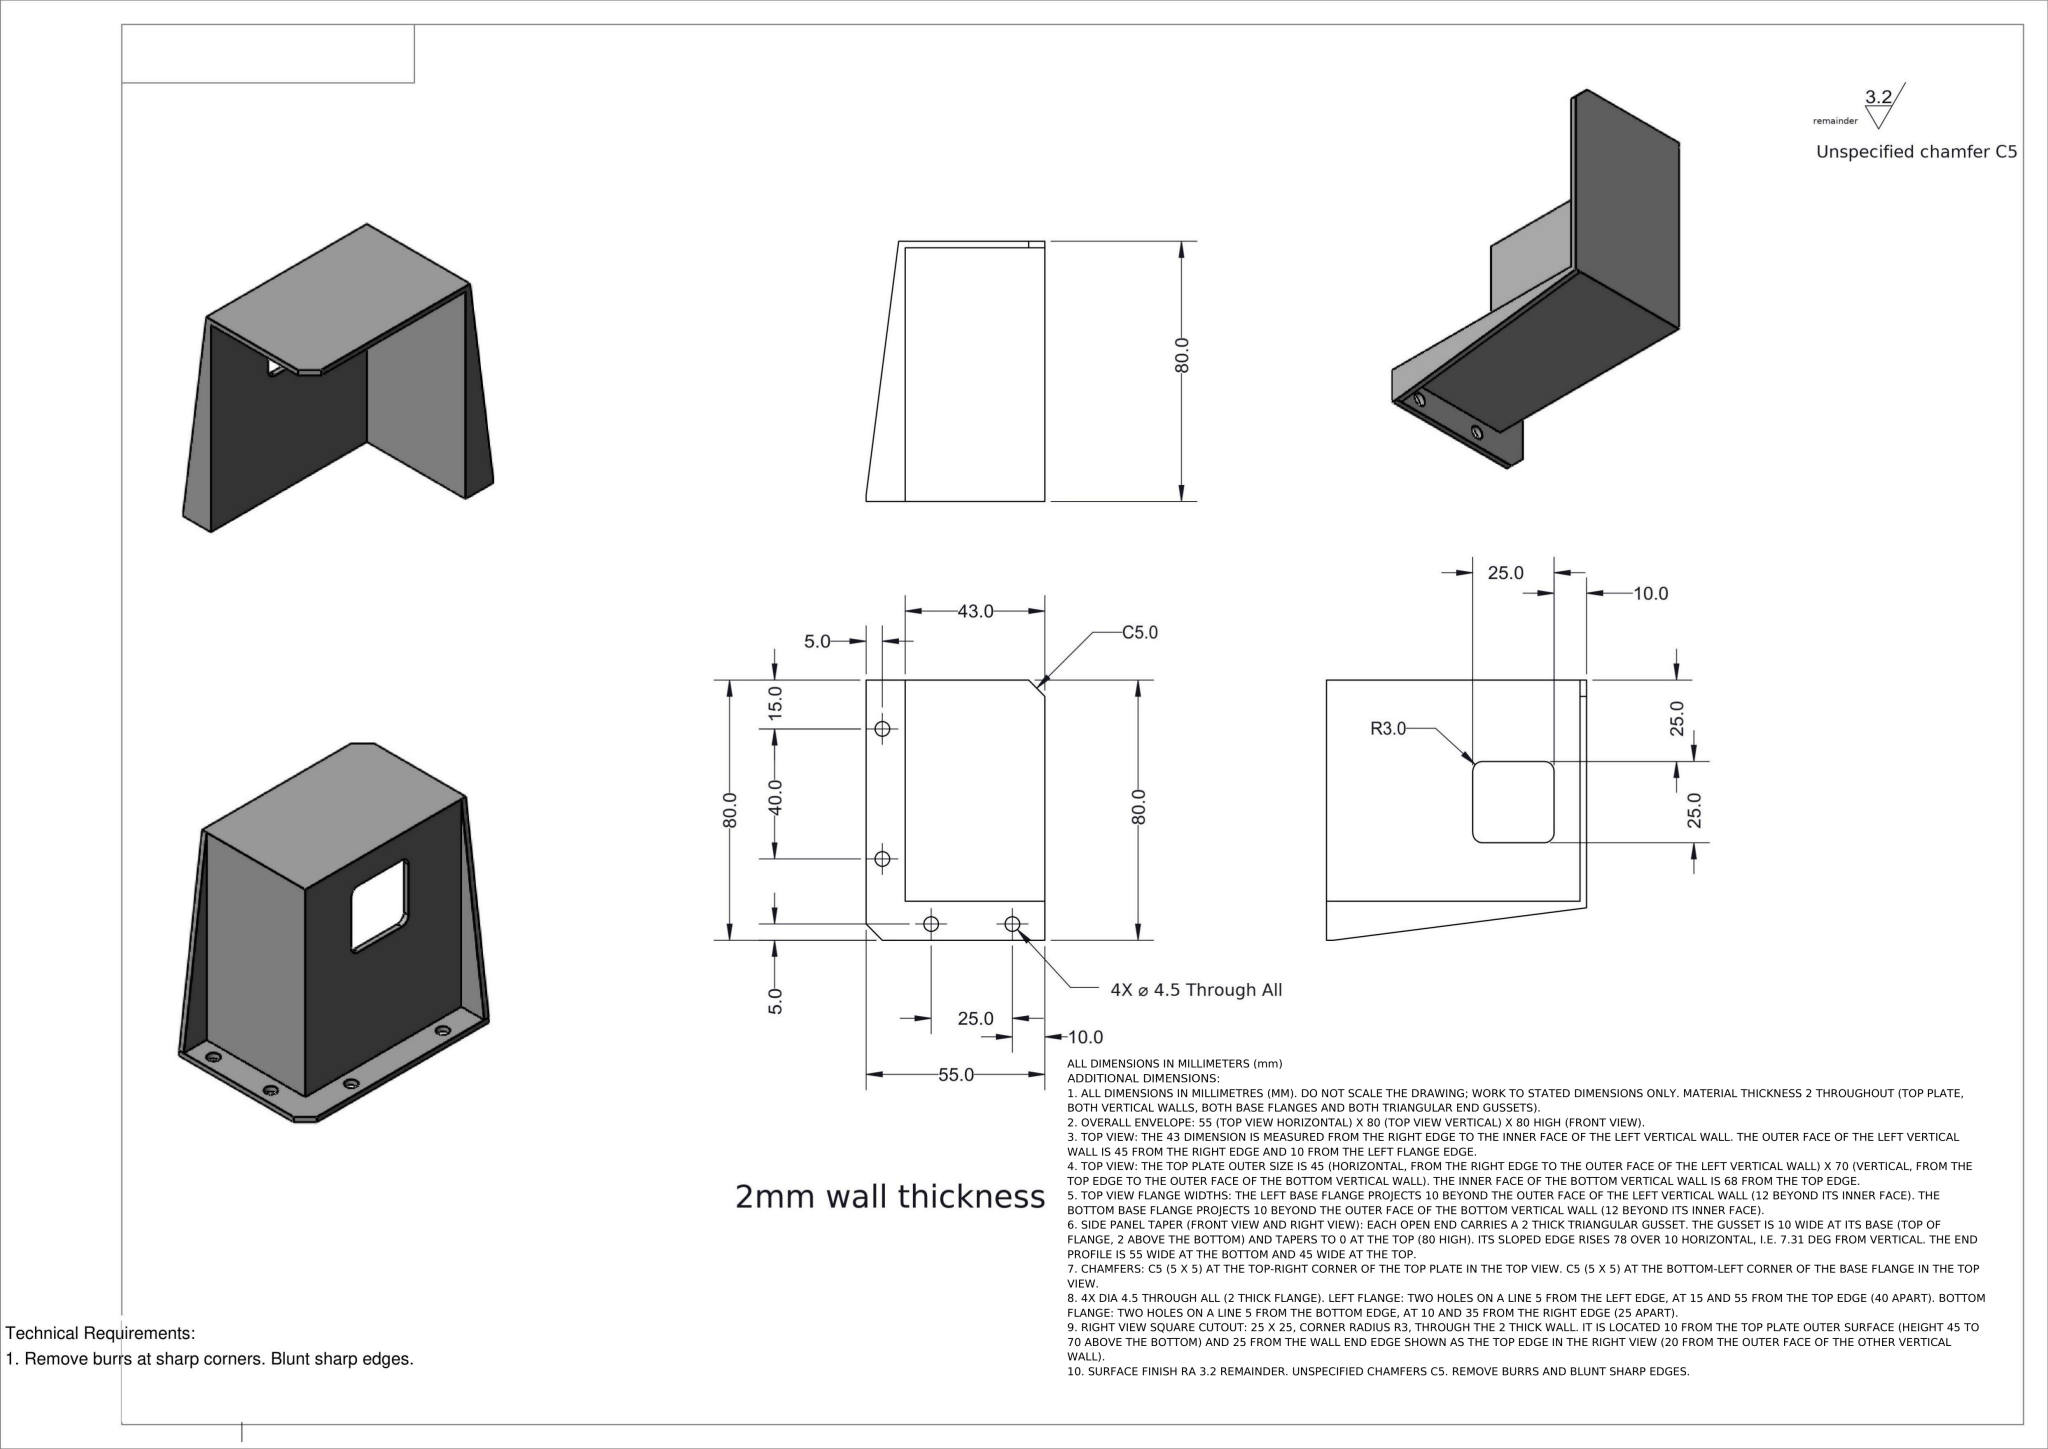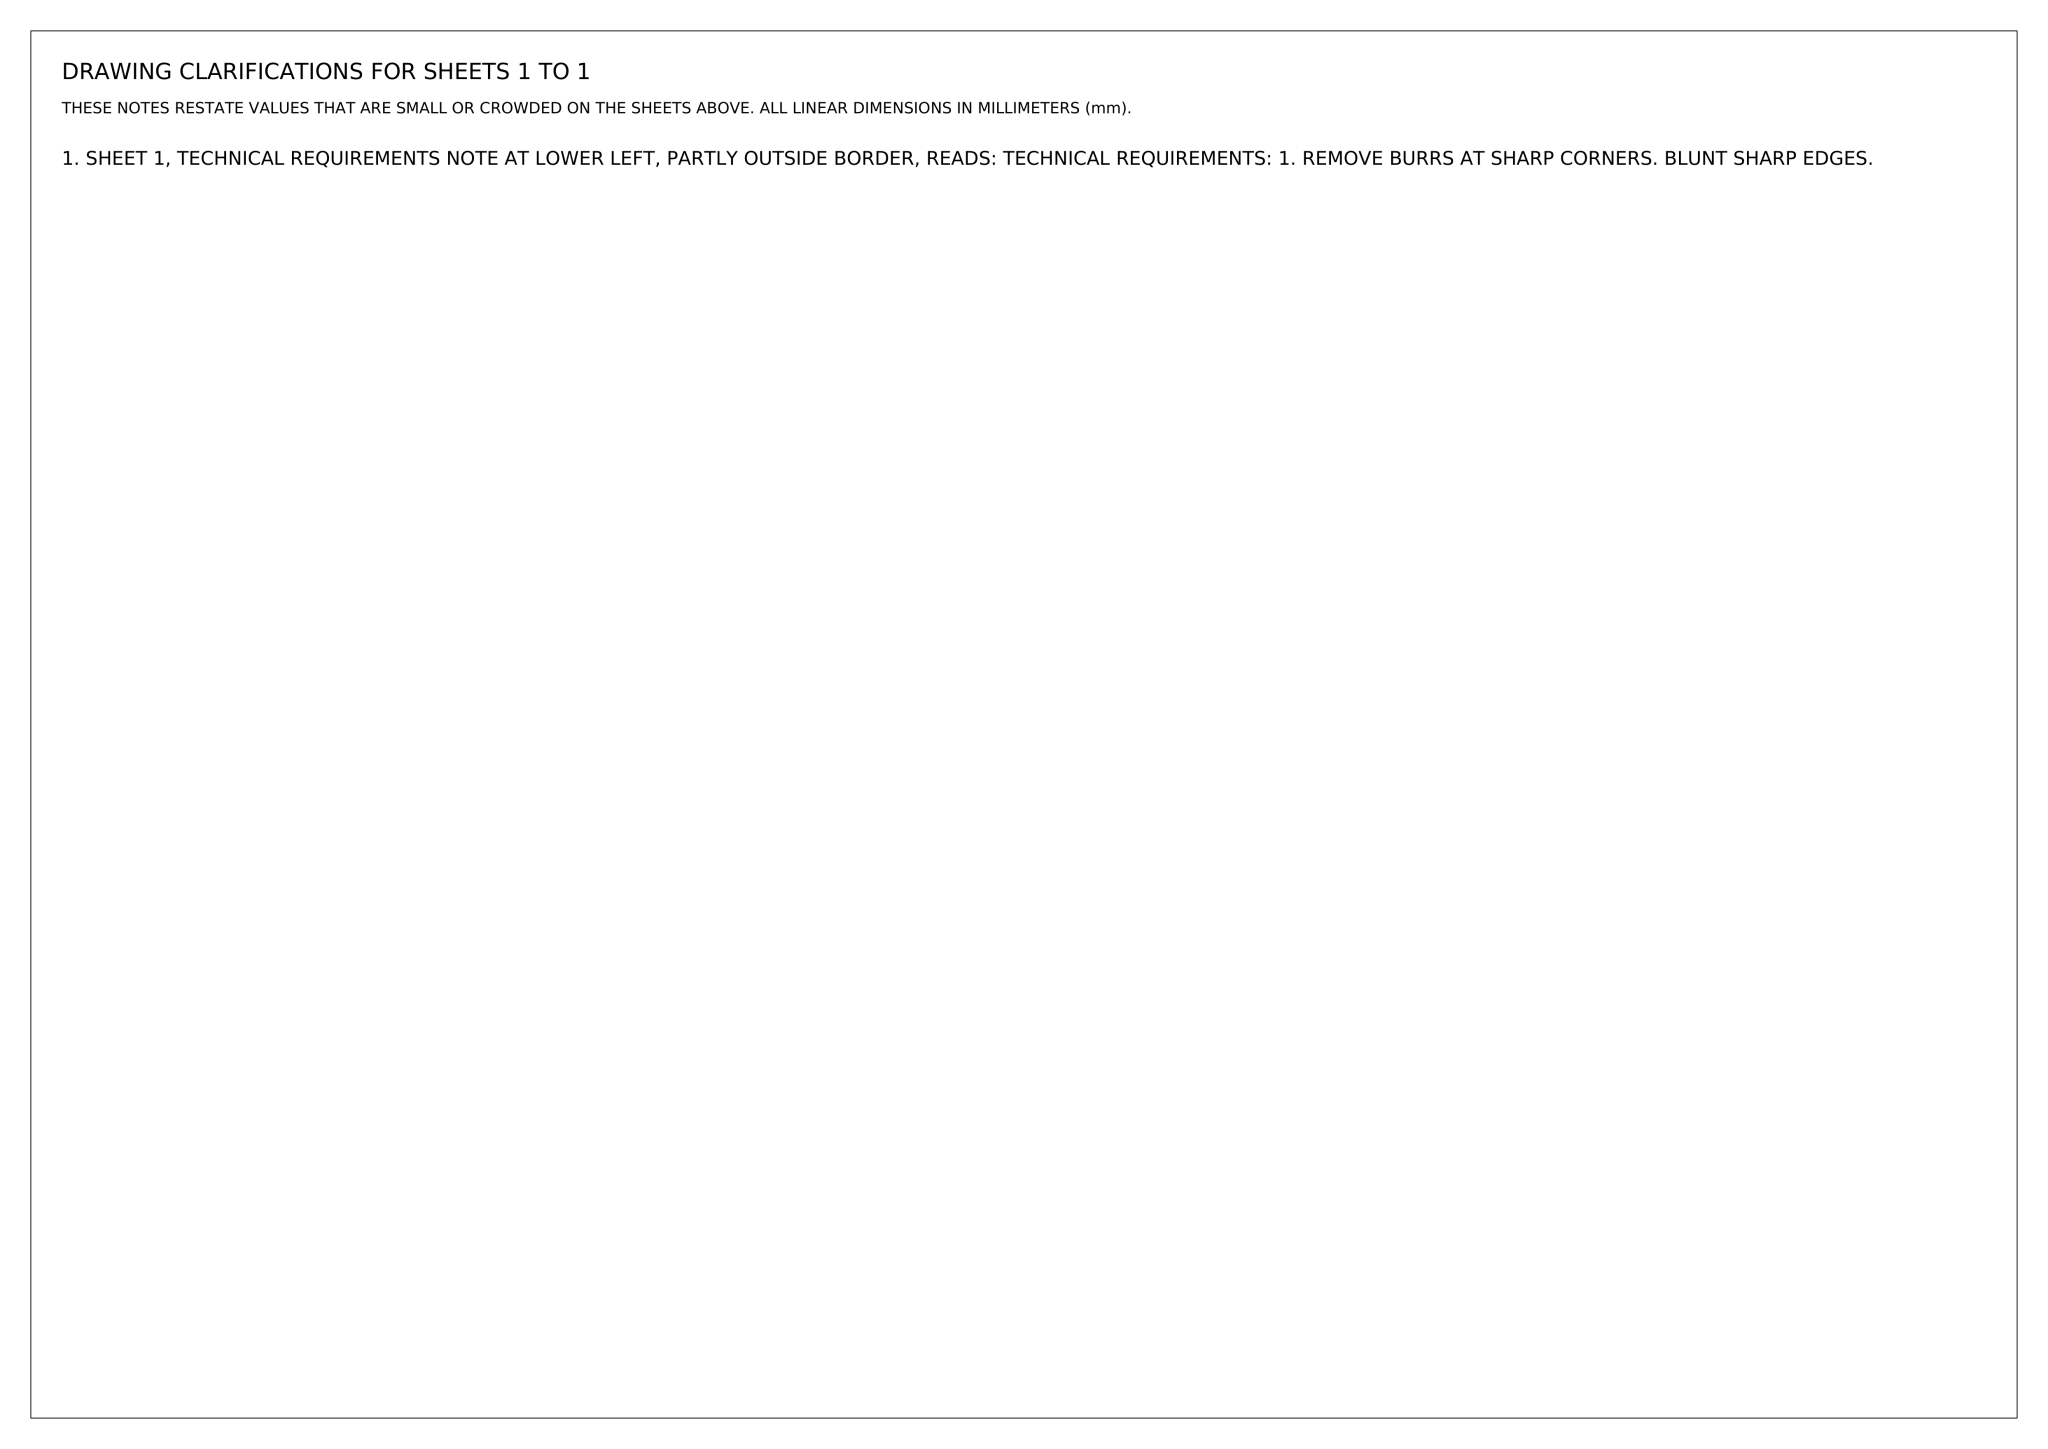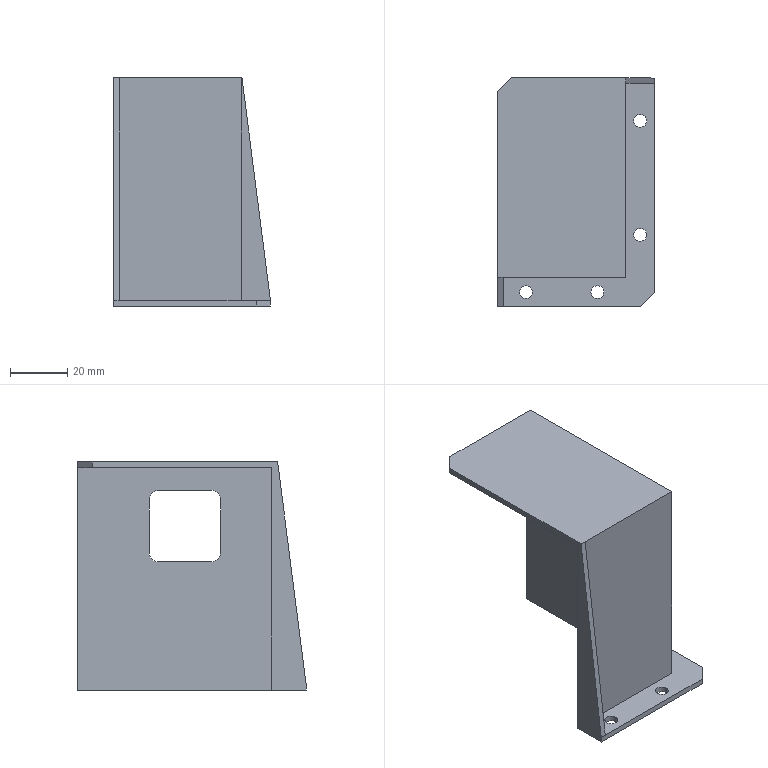Part | NX | mm | 1 solid | 34 faces | box 55 x 80 x 80 mm | volume 26576 mm3 | plane 22 | cylinder 12 | commonest cylinder face diameters 4.5 x8 6 x4